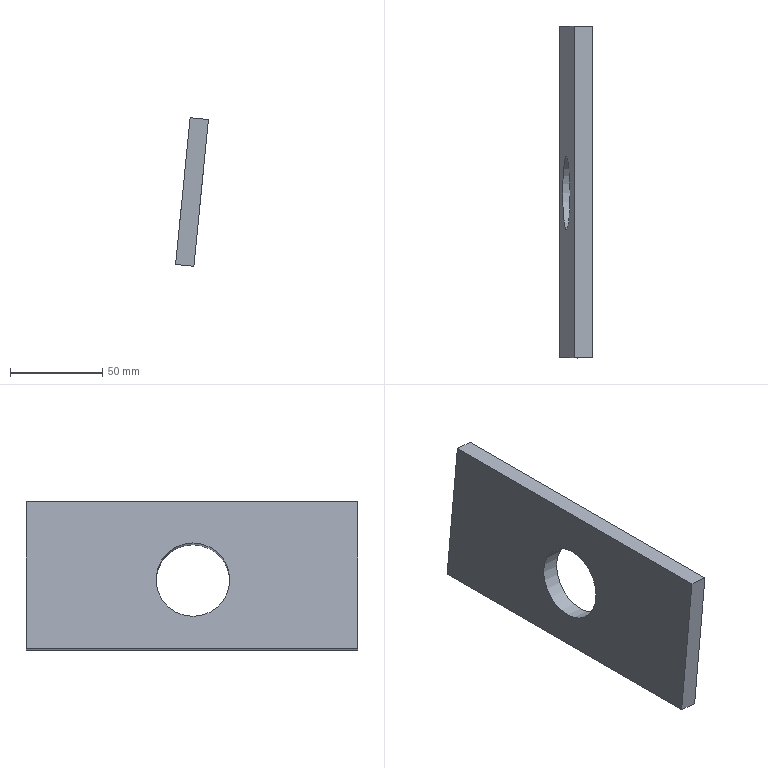Component | NX | UP_FRAME_BLOCK_1 | 1 solid | 7 faces | box 17.9 x 180 x 80.6 mm | volume 131434 mm3 | plane 6 | cylinder 1 | commonest cylinder face diameters 40 x1
STEP:
#1=CARTESIAN_POINT('',(0.,0.,0.));
#2=DIRECTION('',(0.,0.,1.));
#3=DIRECTION('',(1.,0.,0.));
#4=AXIS2_PLACEMENT_3D('',#1,#2,#3);
#5=CARTESIAN_POINT('',(1554.12,-22.,442.548));
#6=VERTEX_POINT('',#5);
#7=CARTESIAN_POINT('',(1546.175,-22.,362.943));
#8=VERTEX_POINT('',#7);
#9=CARTESIAN_POINT('',(1554.12,-22.,442.548));
#10=DIRECTION('',(-0.09932,0.,-0.9951));
#11=VECTOR('',#10,1.);
#12=LINE('',#9,#11);
#13=CARTESIAN_POINT('',(1564.071,-22.,441.554));
#14=DIRECTION('',(0.,1.,0.));
#15=DIRECTION('',(0.09932,0.,0.9951));
#16=AXIS2_PLACEMENT_3D('',#13,#14,#15);
#17=PLANE('',#16);
#18=CARTESIAN_POINT('',(-0.,-10.));
#19=DIRECTION('',(-1.,0.));
#20=VECTOR('',#19,1.);
#21=LINE('',#18,#20);
#22=(GEOMETRIC_REPRESENTATION_CONTEXT(2)PARAMETRIC_REPRESENTATION_CONTEXT()REPRESENTATION_CONTEXT('',''));
#23=DEFINITIONAL_REPRESENTATION('',(#21),#22);
#24=PCURVE('',#17,#23);
#25=CARTESIAN_POINT('',(1546.175,-22.,362.943));
#26=DIRECTION('',(0.9951,0.,-0.09932));
#27=DIRECTION('',(-0.09932,0.,-0.9951));
#28=AXIS2_PLACEMENT_3D('',#25,#26,#27);
#29=PLANE('',#28);
#30=CARTESIAN_POINT('',(-80.,0.));
#31=DIRECTION('',(1.,0.));
#32=VECTOR('',#31,1.);
#33=LINE('',#30,#32);
#34=(GEOMETRIC_REPRESENTATION_CONTEXT(2)PARAMETRIC_REPRESENTATION_CONTEXT()REPRESENTATION_CONTEXT('',''));
#35=DEFINITIONAL_REPRESENTATION('',(#33),#34);
#36=PCURVE('',#29,#35);
#37=SURFACE_CURVE('',#12,(#24,#36),.PCURVE_S1.);
#38=EDGE_CURVE('',#6,#8,#37,.T.);
#39=ORIENTED_EDGE('',*,*,#38,.T.);
#40=CARTESIAN_POINT('',(1556.125,-22.,361.95));
#41=VERTEX_POINT('',#40);
#42=CARTESIAN_POINT('',(1556.125,-22.,361.95));
#43=DIRECTION('',(-0.9951,0.,0.09932));
#44=VECTOR('',#43,1.);
#45=LINE('',#42,#44);
#46=CARTESIAN_POINT('',(-80.,0.));
#47=DIRECTION('',(-0.,-1.));
#48=VECTOR('',#47,1.);
#49=LINE('',#46,#48);
#50=(GEOMETRIC_REPRESENTATION_CONTEXT(2)PARAMETRIC_REPRESENTATION_CONTEXT()REPRESENTATION_CONTEXT('',''));
#51=DEFINITIONAL_REPRESENTATION('',(#49),#50);
#52=PCURVE('',#17,#51);
#53=CARTESIAN_POINT('',(1556.125,-22.,361.95));
#54=DIRECTION('',(0.09932,0.,0.9951));
#55=DIRECTION('',(0.9951,0.,-0.09932));
#56=AXIS2_PLACEMENT_3D('',#53,#54,#55);
#57=PLANE('',#56);
#58=CARTESIAN_POINT('',(0.,0.));
#59=DIRECTION('',(-1.,0.));
#60=VECTOR('',#59,1.);
#61=LINE('',#58,#60);
#62=(GEOMETRIC_REPRESENTATION_CONTEXT(2)PARAMETRIC_REPRESENTATION_CONTEXT()REPRESENTATION_CONTEXT('',''));
#63=DEFINITIONAL_REPRESENTATION('',(#61),#62);
#64=PCURVE('',#57,#63);
#65=SURFACE_CURVE('',#45,(#52,#64),.PCURVE_S1.);
#66=EDGE_CURVE('',#41,#8,#65,.T.);
#67=ORIENTED_EDGE('',*,*,#66,.F.);
#68=CARTESIAN_POINT('',(1564.071,-22.,441.554));
#69=VERTEX_POINT('',#68);
#70=CARTESIAN_POINT('',(1564.071,-22.,441.554));
#71=DIRECTION('',(-0.09932,0.,-0.9951));
#72=VECTOR('',#71,1.);
#73=LINE('',#70,#72);
#74=CARTESIAN_POINT('',(0.,0.));
#75=DIRECTION('',(-1.,0.));
#76=VECTOR('',#75,1.);
#77=LINE('',#74,#76);
#78=(GEOMETRIC_REPRESENTATION_CONTEXT(2)PARAMETRIC_REPRESENTATION_CONTEXT()REPRESENTATION_CONTEXT('',''));
#79=DEFINITIONAL_REPRESENTATION('',(#77),#78);
#80=PCURVE('',#17,#79);
#81=CARTESIAN_POINT('',(1556.125,-22.,361.95));
#82=DIRECTION('',(0.9951,0.,-0.09932));
#83=DIRECTION('',(-0.09932,0.,-0.9951));
#84=AXIS2_PLACEMENT_3D('',#81,#82,#83);
#85=PLANE('',#84);
#86=CARTESIAN_POINT('',(-80.,0.));
#87=DIRECTION('',(1.,0.));
#88=VECTOR('',#87,1.);
#89=LINE('',#86,#88);
#90=(GEOMETRIC_REPRESENTATION_CONTEXT(2)PARAMETRIC_REPRESENTATION_CONTEXT()REPRESENTATION_CONTEXT('',''));
#91=DEFINITIONAL_REPRESENTATION('',(#89),#90);
#92=PCURVE('',#85,#91);
#93=SURFACE_CURVE('',#73,(#80,#92),.PCURVE_S1.);
#94=EDGE_CURVE('',#69,#41,#93,.T.);
#95=ORIENTED_EDGE('',*,*,#94,.F.);
#96=CARTESIAN_POINT('',(1564.071,-22.,441.554));
#97=DIRECTION('',(-0.9951,0.,0.09932));
#98=VECTOR('',#97,1.);
#99=LINE('',#96,#98);
#100=CARTESIAN_POINT('',(0.,0.));
#101=DIRECTION('',(-0.,-1.));
#102=VECTOR('',#101,1.);
#103=LINE('',#100,#102);
#104=(GEOMETRIC_REPRESENTATION_CONTEXT(2)PARAMETRIC_REPRESENTATION_CONTEXT()REPRESENTATION_CONTEXT('',''));
#105=DEFINITIONAL_REPRESENTATION('',(#103),#104);
#106=PCURVE('',#17,#105);
#107=CARTESIAN_POINT('',(1564.071,158.,441.554));
#108=DIRECTION('',(-0.09932,0.,-0.9951));
#109=DIRECTION('',(-0.9951,0.,0.09932));
#110=AXIS2_PLACEMENT_3D('',#107,#108,#109);
#111=PLANE('',#110);
#112=CARTESIAN_POINT('',(0.,-180.));
#113=DIRECTION('',(1.,0.));
#114=VECTOR('',#113,1.);
#115=LINE('',#112,#114);
#116=(GEOMETRIC_REPRESENTATION_CONTEXT(2)PARAMETRIC_REPRESENTATION_CONTEXT()REPRESENTATION_CONTEXT('',''));
#117=DEFINITIONAL_REPRESENTATION('',(#115),#116);
#118=PCURVE('',#111,#117);
#119=SURFACE_CURVE('',#99,(#106,#118),.PCURVE_S1.);
#120=EDGE_CURVE('',#69,#6,#119,.T.);
#121=ORIENTED_EDGE('',*,*,#120,.T.);
#122=EDGE_LOOP('',(#39,#67,#95,#121));
#123=FACE_BOUND('',#122,.T.);
#124=ADVANCED_FACE('',(#123),#17,.F.);
#125=CARTESIAN_POINT('',(1546.175,158.,362.943));
#126=VERTEX_POINT('',#125);
#127=CARTESIAN_POINT('',(1546.175,-22.,362.943));
#128=DIRECTION('',(0.,1.,0.));
#129=VECTOR('',#128,1.);
#130=LINE('',#127,#129);
#131=CARTESIAN_POINT('',(-10.,0.));
#132=DIRECTION('',(0.,1.));
#133=VECTOR('',#132,1.);
#134=LINE('',#131,#133);
#135=(GEOMETRIC_REPRESENTATION_CONTEXT(2)PARAMETRIC_REPRESENTATION_CONTEXT()REPRESENTATION_CONTEXT('',''));
#136=DEFINITIONAL_REPRESENTATION('',(#134),#135);
#137=PCURVE('',#57,#136);
#138=CARTESIAN_POINT('',(0.,0.));
#139=DIRECTION('',(0.,1.));
#140=VECTOR('',#139,1.);
#141=LINE('',#138,#140);
#142=(GEOMETRIC_REPRESENTATION_CONTEXT(2)PARAMETRIC_REPRESENTATION_CONTEXT()REPRESENTATION_CONTEXT('',''));
#143=DEFINITIONAL_REPRESENTATION('',(#141),#142);
#144=PCURVE('',#29,#143);
#145=SURFACE_CURVE('',#130,(#137,#144),.PCURVE_S1.);
#146=EDGE_CURVE('',#8,#126,#145,.T.);
#147=ORIENTED_EDGE('',*,*,#146,.T.);
#148=CARTESIAN_POINT('',(1556.125,158.,361.95));
#149=VERTEX_POINT('',#148);
#150=CARTESIAN_POINT('',(1556.125,158.,361.95));
#151=DIRECTION('',(-0.9951,0.,0.09932));
#152=VECTOR('',#151,1.);
#153=LINE('',#150,#152);
#154=CARTESIAN_POINT('',(0.,180.));
#155=DIRECTION('',(-1.,0.));
#156=VECTOR('',#155,1.);
#157=LINE('',#154,#156);
#158=(GEOMETRIC_REPRESENTATION_CONTEXT(2)PARAMETRIC_REPRESENTATION_CONTEXT()REPRESENTATION_CONTEXT('',''));
#159=DEFINITIONAL_REPRESENTATION('',(#157),#158);
#160=PCURVE('',#57,#159);
#161=CARTESIAN_POINT('',(1556.125,158.,361.95));
#162=DIRECTION('',(0.,-1.,0.));
#163=DIRECTION('',(-0.09932,0.,-0.9951));
#164=AXIS2_PLACEMENT_3D('',#161,#162,#163);
#165=PLANE('',#164);
#166=CARTESIAN_POINT('',(0.,0.));
#167=DIRECTION('',(0.,-1.));
#168=VECTOR('',#167,1.);
#169=LINE('',#166,#168);
#170=(GEOMETRIC_REPRESENTATION_CONTEXT(2)PARAMETRIC_REPRESENTATION_CONTEXT()REPRESENTATION_CONTEXT('',''));
#171=DEFINITIONAL_REPRESENTATION('',(#169),#170);
#172=PCURVE('',#165,#171);
#173=SURFACE_CURVE('',#153,(#160,#172),.PCURVE_S1.);
#174=EDGE_CURVE('',#149,#126,#173,.T.);
#175=ORIENTED_EDGE('',*,*,#174,.F.);
#176=CARTESIAN_POINT('',(1556.125,-22.,361.95));
#177=DIRECTION('',(0.,1.,0.));
#178=VECTOR('',#177,1.);
#179=LINE('',#176,#178);
#180=CARTESIAN_POINT('',(0.,0.));
#181=DIRECTION('',(0.,1.));
#182=VECTOR('',#181,1.);
#183=LINE('',#180,#182);
#184=(GEOMETRIC_REPRESENTATION_CONTEXT(2)PARAMETRIC_REPRESENTATION_CONTEXT()REPRESENTATION_CONTEXT('',''));
#185=DEFINITIONAL_REPRESENTATION('',(#183),#184);
#186=PCURVE('',#57,#185);
#187=CARTESIAN_POINT('',(0.,0.));
#188=DIRECTION('',(0.,1.));
#189=VECTOR('',#188,1.);
#190=LINE('',#187,#189);
#191=(GEOMETRIC_REPRESENTATION_CONTEXT(2)PARAMETRIC_REPRESENTATION_CONTEXT()REPRESENTATION_CONTEXT('',''));
#192=DEFINITIONAL_REPRESENTATION('',(#190),#191);
#193=PCURVE('',#85,#192);
#194=SURFACE_CURVE('',#179,(#186,#193),.PCURVE_S1.);
#195=EDGE_CURVE('',#41,#149,#194,.T.);
#196=ORIENTED_EDGE('',*,*,#195,.F.);
#197=ORIENTED_EDGE('',*,*,#66,.T.);
#198=EDGE_LOOP('',(#147,#175,#196,#197));
#199=FACE_BOUND('',#198,.T.);
#200=ADVANCED_FACE('',(#199),#57,.F.);
#201=CARTESIAN_POINT('',(1554.12,158.,442.548));
#202=VERTEX_POINT('',#201);
#203=CARTESIAN_POINT('',(1546.175,158.,362.943));
#204=DIRECTION('',(0.09932,0.,0.9951));
#205=VECTOR('',#204,1.);
#206=LINE('',#203,#205);
#207=CARTESIAN_POINT('',(0.,-10.));
#208=DIRECTION('',(-1.,-0.));
#209=VECTOR('',#208,1.);
#210=LINE('',#207,#209);
#211=(GEOMETRIC_REPRESENTATION_CONTEXT(2)PARAMETRIC_REPRESENTATION_CONTEXT()REPRESENTATION_CONTEXT('',''));
#212=DEFINITIONAL_REPRESENTATION('',(#210),#211);
#213=PCURVE('',#165,#212);
#214=CARTESIAN_POINT('',(0.,180.));
#215=DIRECTION('',(-1.,0.));
#216=VECTOR('',#215,1.);
#217=LINE('',#214,#216);
#218=(GEOMETRIC_REPRESENTATION_CONTEXT(2)PARAMETRIC_REPRESENTATION_CONTEXT()REPRESENTATION_CONTEXT('',''));
#219=DEFINITIONAL_REPRESENTATION('',(#217),#218);
#220=PCURVE('',#29,#219);
#221=SURFACE_CURVE('',#206,(#213,#220),.PCURVE_S1.);
#222=EDGE_CURVE('',#126,#202,#221,.T.);
#223=ORIENTED_EDGE('',*,*,#222,.T.);
#224=CARTESIAN_POINT('',(1564.071,158.,441.554));
#225=VERTEX_POINT('',#224);
#226=CARTESIAN_POINT('',(1564.071,158.,441.554));
#227=DIRECTION('',(-0.9951,0.,0.09932));
#228=VECTOR('',#227,1.);
#229=LINE('',#226,#228);
#230=CARTESIAN_POINT('',(-80.,-0.));
#231=DIRECTION('',(0.,-1.));
#232=VECTOR('',#231,1.);
#233=LINE('',#230,#232);
#234=(GEOMETRIC_REPRESENTATION_CONTEXT(2)PARAMETRIC_REPRESENTATION_CONTEXT()REPRESENTATION_CONTEXT('',''));
#235=DEFINITIONAL_REPRESENTATION('',(#233),#234);
#236=PCURVE('',#165,#235);
#237=CARTESIAN_POINT('',(0.,0.));
#238=DIRECTION('',(1.,0.));
#239=VECTOR('',#238,1.);
#240=LINE('',#237,#239);
#241=(GEOMETRIC_REPRESENTATION_CONTEXT(2)PARAMETRIC_REPRESENTATION_CONTEXT()REPRESENTATION_CONTEXT('',''));
#242=DEFINITIONAL_REPRESENTATION('',(#240),#241);
#243=PCURVE('',#111,#242);
#244=SURFACE_CURVE('',#229,(#236,#243),.PCURVE_S1.);
#245=EDGE_CURVE('',#225,#202,#244,.T.);
#246=ORIENTED_EDGE('',*,*,#245,.F.);
#247=CARTESIAN_POINT('',(1556.125,158.,361.95));
#248=DIRECTION('',(0.09932,0.,0.9951));
#249=VECTOR('',#248,1.);
#250=LINE('',#247,#249);
#251=CARTESIAN_POINT('',(0.,0.));
#252=DIRECTION('',(-1.,-0.));
#253=VECTOR('',#252,1.);
#254=LINE('',#251,#253);
#255=(GEOMETRIC_REPRESENTATION_CONTEXT(2)PARAMETRIC_REPRESENTATION_CONTEXT()REPRESENTATION_CONTEXT('',''));
#256=DEFINITIONAL_REPRESENTATION('',(#254),#255);
#257=PCURVE('',#165,#256);
#258=CARTESIAN_POINT('',(0.,180.));
#259=DIRECTION('',(-1.,0.));
#260=VECTOR('',#259,1.);
#261=LINE('',#258,#260);
#262=(GEOMETRIC_REPRESENTATION_CONTEXT(2)PARAMETRIC_REPRESENTATION_CONTEXT()REPRESENTATION_CONTEXT('',''));
#263=DEFINITIONAL_REPRESENTATION('',(#261),#262);
#264=PCURVE('',#85,#263);
#265=SURFACE_CURVE('',#250,(#257,#264),.PCURVE_S1.);
#266=EDGE_CURVE('',#149,#225,#265,.T.);
#267=ORIENTED_EDGE('',*,*,#266,.F.);
#268=ORIENTED_EDGE('',*,*,#174,.T.);
#269=EDGE_LOOP('',(#223,#246,#267,#268));
#270=FACE_BOUND('',#269,.T.);
#271=ADVANCED_FACE('',(#270),#165,.F.);
#272=CARTESIAN_POINT('',(1554.12,158.,442.548));
#273=DIRECTION('',(0.,-1.,0.));
#274=VECTOR('',#273,1.);
#275=LINE('',#272,#274);
#276=CARTESIAN_POINT('',(10.,0.));
#277=DIRECTION('',(0.,-1.));
#278=VECTOR('',#277,1.);
#279=LINE('',#276,#278);
#280=(GEOMETRIC_REPRESENTATION_CONTEXT(2)PARAMETRIC_REPRESENTATION_CONTEXT()REPRESENTATION_CONTEXT('',''));
#281=DEFINITIONAL_REPRESENTATION('',(#279),#280);
#282=PCURVE('',#111,#281);
#283=CARTESIAN_POINT('',(-80.,180.));
#284=DIRECTION('',(0.,-1.));
#285=VECTOR('',#284,1.);
#286=LINE('',#283,#285);
#287=(GEOMETRIC_REPRESENTATION_CONTEXT(2)PARAMETRIC_REPRESENTATION_CONTEXT()REPRESENTATION_CONTEXT('',''));
#288=DEFINITIONAL_REPRESENTATION('',(#286),#287);
#289=PCURVE('',#29,#288);
#290=SURFACE_CURVE('',#275,(#282,#289),.PCURVE_S1.);
#291=EDGE_CURVE('',#202,#6,#290,.T.);
#292=ORIENTED_EDGE('',*,*,#291,.T.);
#293=ORIENTED_EDGE('',*,*,#120,.F.);
#294=CARTESIAN_POINT('',(1564.071,158.,441.554));
#295=DIRECTION('',(0.,-1.,0.));
#296=VECTOR('',#295,1.);
#297=LINE('',#294,#296);
#298=CARTESIAN_POINT('',(0.,0.));
#299=DIRECTION('',(0.,-1.));
#300=VECTOR('',#299,1.);
#301=LINE('',#298,#300);
#302=(GEOMETRIC_REPRESENTATION_CONTEXT(2)PARAMETRIC_REPRESENTATION_CONTEXT()REPRESENTATION_CONTEXT('',''));
#303=DEFINITIONAL_REPRESENTATION('',(#301),#302);
#304=PCURVE('',#111,#303);
#305=CARTESIAN_POINT('',(-80.,180.));
#306=DIRECTION('',(0.,-1.));
#307=VECTOR('',#306,1.);
#308=LINE('',#305,#307);
#309=(GEOMETRIC_REPRESENTATION_CONTEXT(2)PARAMETRIC_REPRESENTATION_CONTEXT()REPRESENTATION_CONTEXT('',''));
#310=DEFINITIONAL_REPRESENTATION('',(#308),#309);
#311=PCURVE('',#85,#310);
#312=SURFACE_CURVE('',#297,(#304,#311),.PCURVE_S1.);
#313=EDGE_CURVE('',#225,#69,#312,.T.);
#314=ORIENTED_EDGE('',*,*,#313,.F.);
#315=ORIENTED_EDGE('',*,*,#245,.T.);
#316=EDGE_LOOP('',(#292,#293,#314,#315));
#317=FACE_BOUND('',#316,.T.);
#318=ADVANCED_FACE('',(#317),#111,.F.);
#319=CARTESIAN_POINT('',(1557.864,67.5,379.363));
#320=VERTEX_POINT('',#319);
#321=CARTESIAN_POINT('',(1559.85,67.5,399.265));
#322=DIRECTION('',(0.9951,0.,-0.09932));
#323=DIRECTION('',(-0.09932,0.,-0.9951));
#324=AXIS2_PLACEMENT_3D('',#321,#322,#323);
#325=CIRCLE('',#324,20.);
#326=CARTESIAN_POINT('',(-37.5,89.5));
#327=DIRECTION('',(1.,0.));
#328=AXIS2_PLACEMENT_2D('',#326,#327);
#329=CIRCLE('',#328,20.);
#330=(GEOMETRIC_REPRESENTATION_CONTEXT(2)PARAMETRIC_REPRESENTATION_CONTEXT()REPRESENTATION_CONTEXT('',''));
#331=DEFINITIONAL_REPRESENTATION('',(#329),#330);
#332=PCURVE('',#85,#331);
#333=CARTESIAN_POINT('',(1544.924,67.5,400.754));
#334=DIRECTION('',(0.9951,0.,-0.09932));
#335=DIRECTION('',(-0.09932,0.,-0.9951));
#336=AXIS2_PLACEMENT_3D('',#333,#334,#335);
#337=CYLINDRICAL_SURFACE('',#336,20.);
#338=CARTESIAN_POINT('',(0.,15.));
#339=DIRECTION('',(1.,0.));
#340=VECTOR('',#339,1.);
#341=LINE('',#338,#340);
#342=(GEOMETRIC_REPRESENTATION_CONTEXT(2)PARAMETRIC_REPRESENTATION_CONTEXT()REPRESENTATION_CONTEXT('',''));
#343=DEFINITIONAL_REPRESENTATION('',(#341),#342);
#344=PCURVE('',#337,#343);
#345=SURFACE_CURVE('',#325,(#332,#344),.PCURVE_S1.);
#346=EDGE_CURVE('',#320,#320,#345,.T.);
#347=ORIENTED_EDGE('',*,*,#346,.F.);
#348=EDGE_LOOP('',(#347));
#349=FACE_BOUND('',#348,.T.);
#350=ORIENTED_EDGE('',*,*,#94,.T.);
#351=ORIENTED_EDGE('',*,*,#195,.T.);
#352=ORIENTED_EDGE('',*,*,#266,.T.);
#353=ORIENTED_EDGE('',*,*,#313,.T.);
#354=EDGE_LOOP('',(#350,#351,#352,#353));
#355=FACE_BOUND('',#354,.T.);
#356=ADVANCED_FACE('',(#349,#355),#85,.T.);
#357=CARTESIAN_POINT('',(1547.913,67.5,380.357));
#358=VERTEX_POINT('',#357);
#359=CARTESIAN_POINT('',(1549.899,67.5,400.258));
#360=DIRECTION('',(0.9951,0.,-0.09932));
#361=DIRECTION('',(-0.09932,0.,-0.9951));
#362=AXIS2_PLACEMENT_3D('',#359,#360,#361);
#363=CIRCLE('',#362,20.);
#364=CARTESIAN_POINT('',(-37.5,89.5));
#365=DIRECTION('',(1.,0.));
#366=AXIS2_PLACEMENT_2D('',#364,#365);
#367=CIRCLE('',#366,20.);
#368=(GEOMETRIC_REPRESENTATION_CONTEXT(2)PARAMETRIC_REPRESENTATION_CONTEXT()REPRESENTATION_CONTEXT('',''));
#369=DEFINITIONAL_REPRESENTATION('',(#367),#368);
#370=PCURVE('',#29,#369);
#371=CARTESIAN_POINT('',(0.,5.));
#372=DIRECTION('',(1.,0.));
#373=VECTOR('',#372,1.);
#374=LINE('',#371,#373);
#375=(GEOMETRIC_REPRESENTATION_CONTEXT(2)PARAMETRIC_REPRESENTATION_CONTEXT()REPRESENTATION_CONTEXT('',''));
#376=DEFINITIONAL_REPRESENTATION('',(#374),#375);
#377=PCURVE('',#337,#376);
#378=SURFACE_CURVE('',#363,(#370,#377),.PCURVE_S1.);
#379=EDGE_CURVE('',#358,#358,#378,.T.);
#380=ORIENTED_EDGE('',*,*,#379,.T.);
#381=EDGE_LOOP('',(#380));
#382=FACE_BOUND('',#381,.T.);
#383=ORIENTED_EDGE('',*,*,#38,.F.);
#384=ORIENTED_EDGE('',*,*,#291,.F.);
#385=ORIENTED_EDGE('',*,*,#222,.F.);
#386=ORIENTED_EDGE('',*,*,#146,.F.);
#387=EDGE_LOOP('',(#383,#384,#385,#386));
#388=FACE_BOUND('',#387,.T.);
#389=ADVANCED_FACE('',(#382,#388),#29,.F.);
#390=ORIENTED_EDGE('',*,*,#346,.F.);
#391=CARTESIAN_POINT('',(1547.913,67.5,380.357));
#392=CARTESIAN_POINT('',(1557.864,67.5,379.363));
#393=B_SPLINE_CURVE_WITH_KNOTS('',1,(#391,#392),.UNSPECIFIED.,.F.,.F.,(2,2),(5.,15.),.PIECEWISE_BEZIER_KNOTS.);
#394=CARTESIAN_POINT('',(0.,0.));
#395=DIRECTION('',(0.,1.));
#396=VECTOR('',#395,1.);
#397=LINE('',#394,#396);
#398=(GEOMETRIC_REPRESENTATION_CONTEXT(2)PARAMETRIC_REPRESENTATION_CONTEXT()REPRESENTATION_CONTEXT('',''));
#399=DEFINITIONAL_REPRESENTATION('',(#397),#398);
#400=PCURVE('',#337,#399);
#401=CARTESIAN_POINT('',(6.283,0.));
#402=DIRECTION('',(0.,1.));
#403=VECTOR('',#402,1.);
#404=LINE('',#401,#403);
#405=(GEOMETRIC_REPRESENTATION_CONTEXT(2)PARAMETRIC_REPRESENTATION_CONTEXT()REPRESENTATION_CONTEXT('',''));
#406=DEFINITIONAL_REPRESENTATION('',(#404),#405);
#407=PCURVE('',#337,#406);
#408=SEAM_CURVE('',#393,(#400,#407),.PCURVE_S1.);
#409=EDGE_CURVE('',#358,#320,#408,.T.);
#410=ORIENTED_EDGE('',*,*,#409,.F.);
#411=ORIENTED_EDGE('',*,*,#379,.T.);
#412=ORIENTED_EDGE('',*,*,#409,.T.);
#413=EDGE_LOOP('',(#390,#410,#411,#412));
#414=FACE_BOUND('',#413,.F.);
#415=ADVANCED_FACE('',(#414),#337,.F.);
#416=CLOSED_SHELL('',(#124,#200,#271,#318,#356,#389,#415));
#417=MANIFOLD_SOLID_BREP('',#416);
#418=(LENGTH_UNIT()NAMED_UNIT(*)SI_UNIT(.MILLI.,.METRE.));
#419=UNCERTAINTY_MEASURE_WITH_UNIT(LENGTH_MEASURE(0.000002),#418,'','');
#420=(NAMED_UNIT(*)PLANE_ANGLE_UNIT()SI_UNIT($,.RADIAN.));
#421=(NAMED_UNIT(*)SI_UNIT($,.STERADIAN.)SOLID_ANGLE_UNIT());
#422=(GEOMETRIC_REPRESENTATION_CONTEXT(3)GLOBAL_UNCERTAINTY_ASSIGNED_CONTEXT((#419))GLOBAL_UNIT_ASSIGNED_CONTEXT((#418,#420,#421))REPRESENTATION_CONTEXT('',''));
#423=ADVANCED_BREP_SHAPE_REPRESENTATION('',(#4,#417),#422);